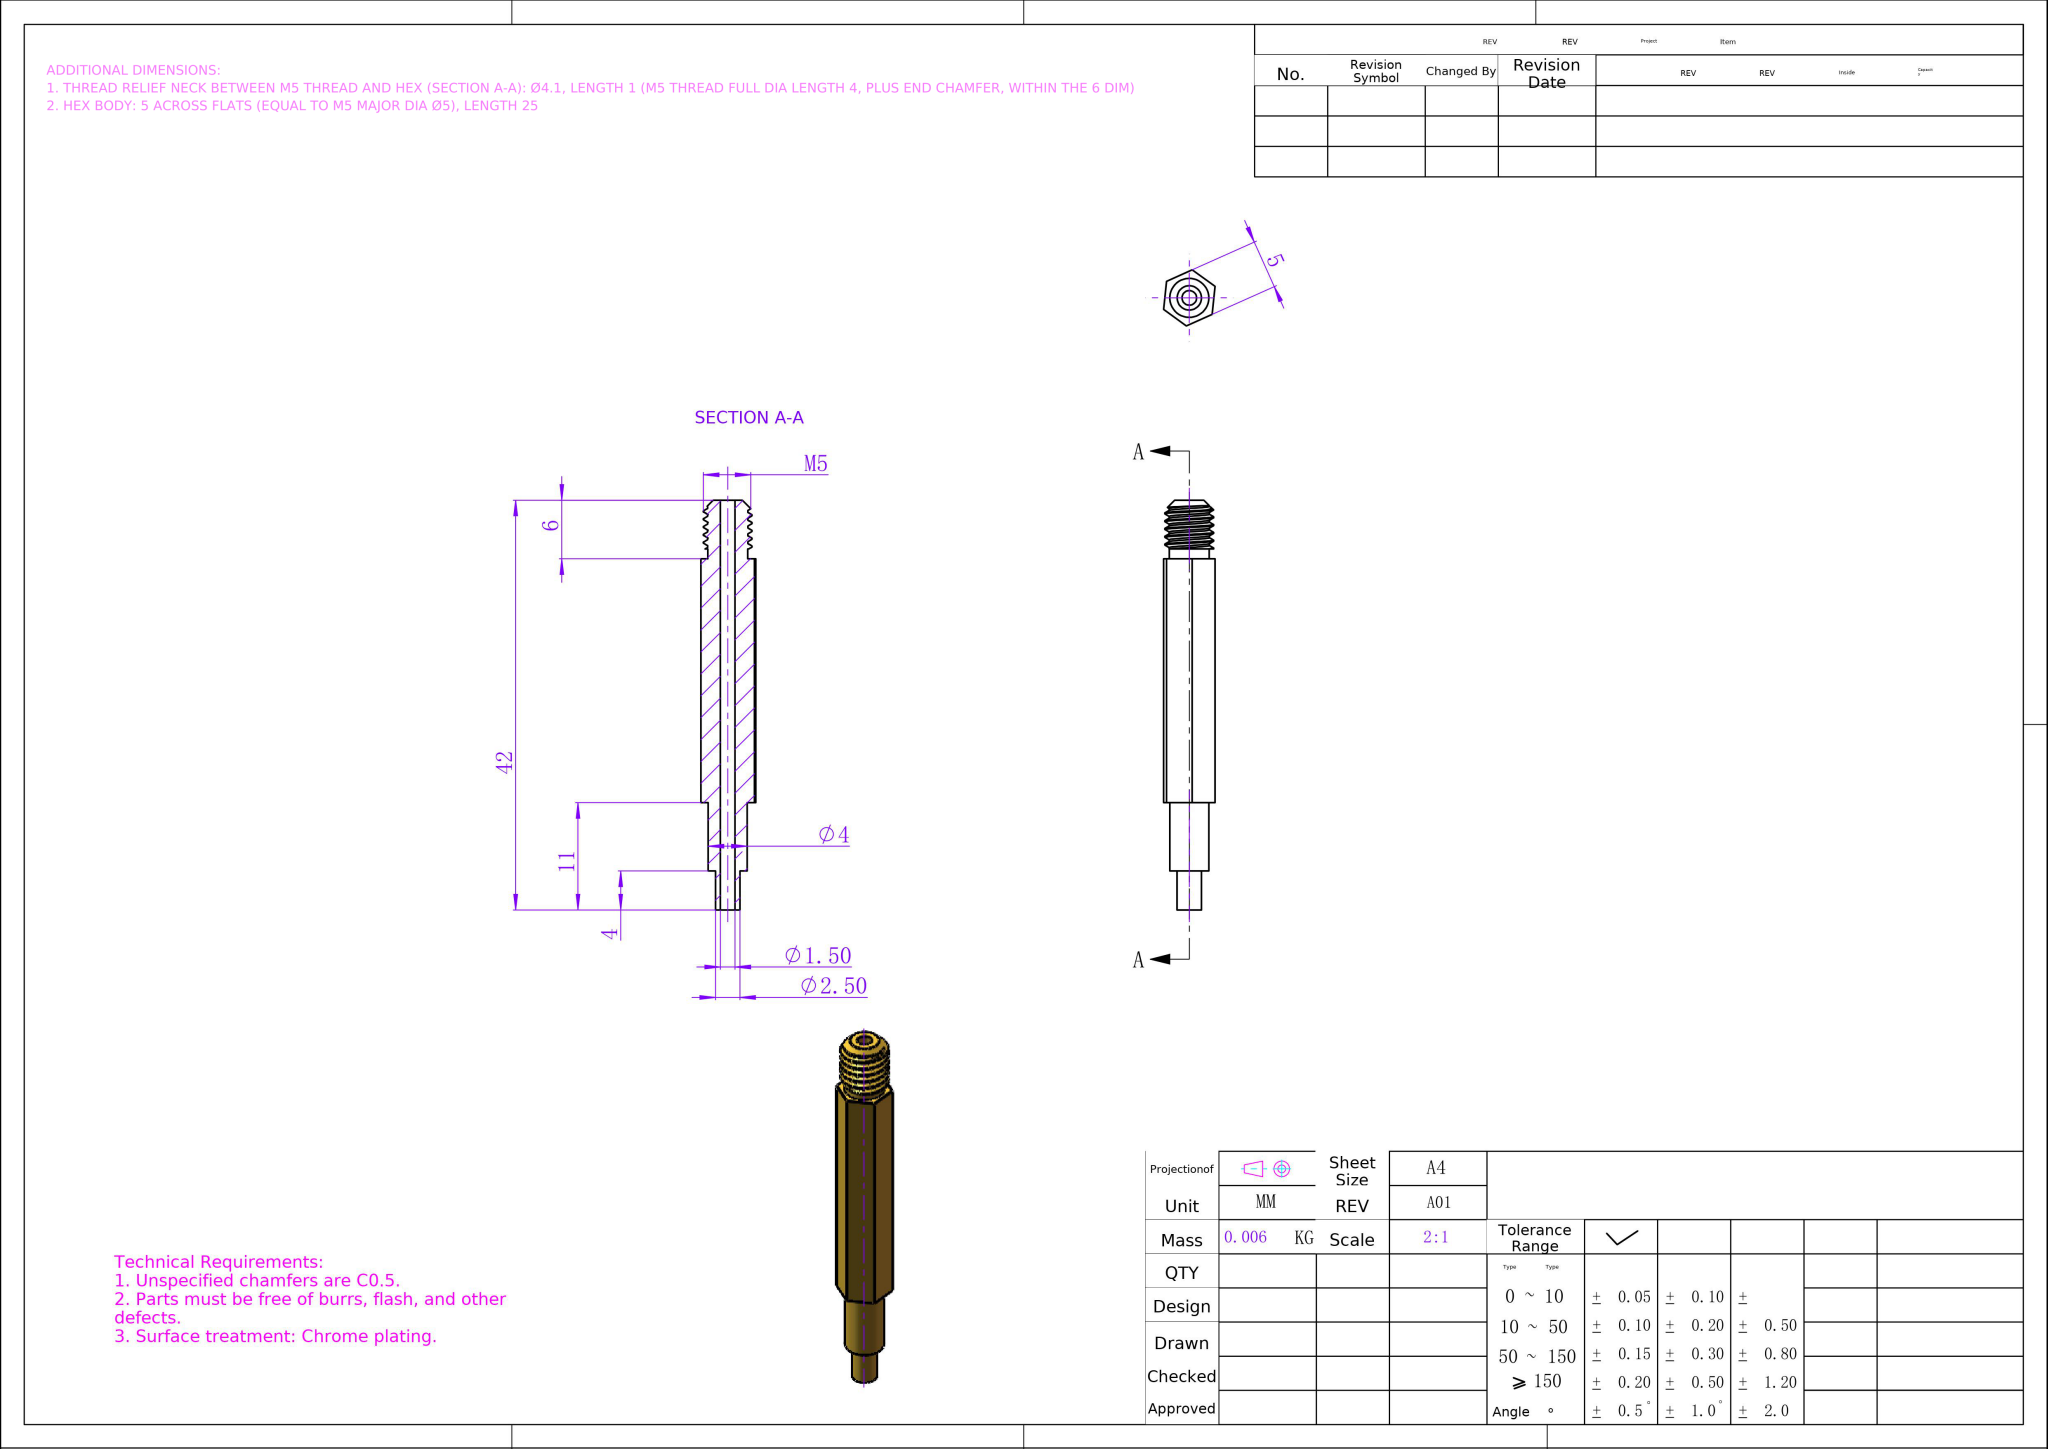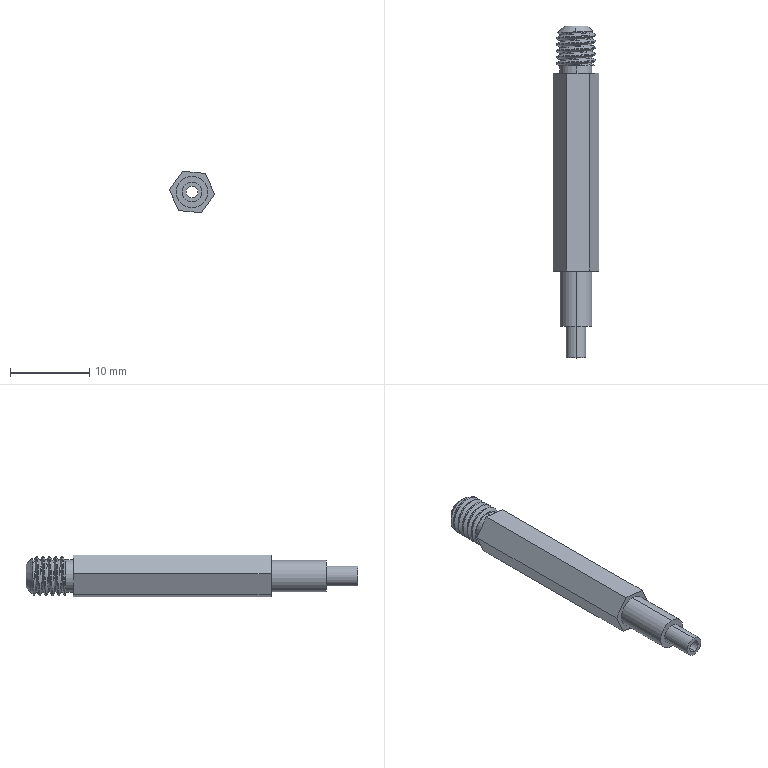Part | NX | mm | 1 solid | 37 faces | box 5.74 x 42 x 5.27 mm | volume 664 mm3 | cylinder 19 | plane 12 | cone 3 | spline 3 | commonest cylinder face diameters 5 x11 4.1 x2 4 x2 2.5 x2 1.5 x2